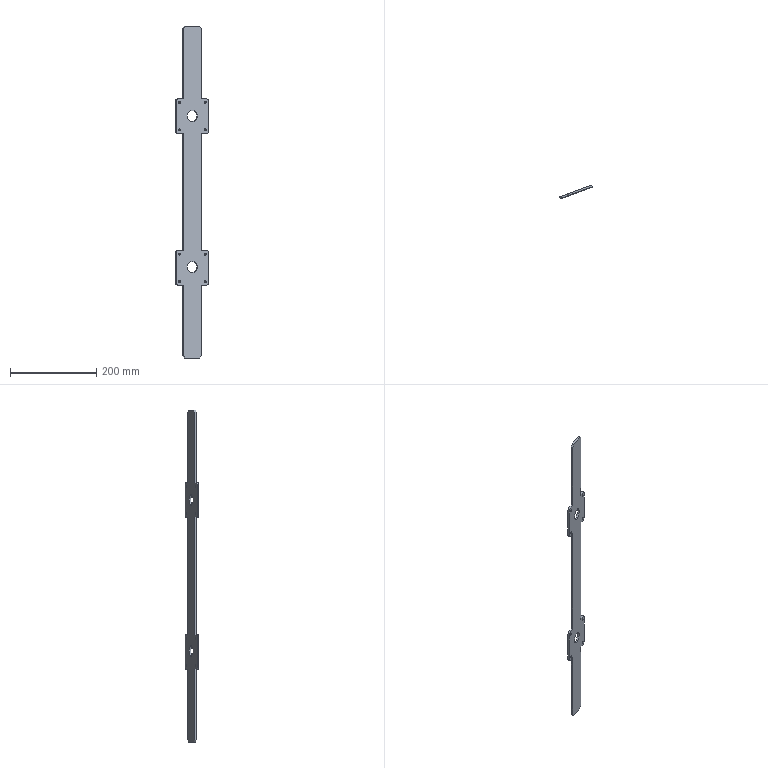Component | SolidWorks | 03-02MotorBracket1-1 | 1 solid | 54 faces | volume 155753 mm3 | cylinder 28 | plane 26 | commonest cylinder face diameters 5 x16 10 x8 26 x4 | material Q235